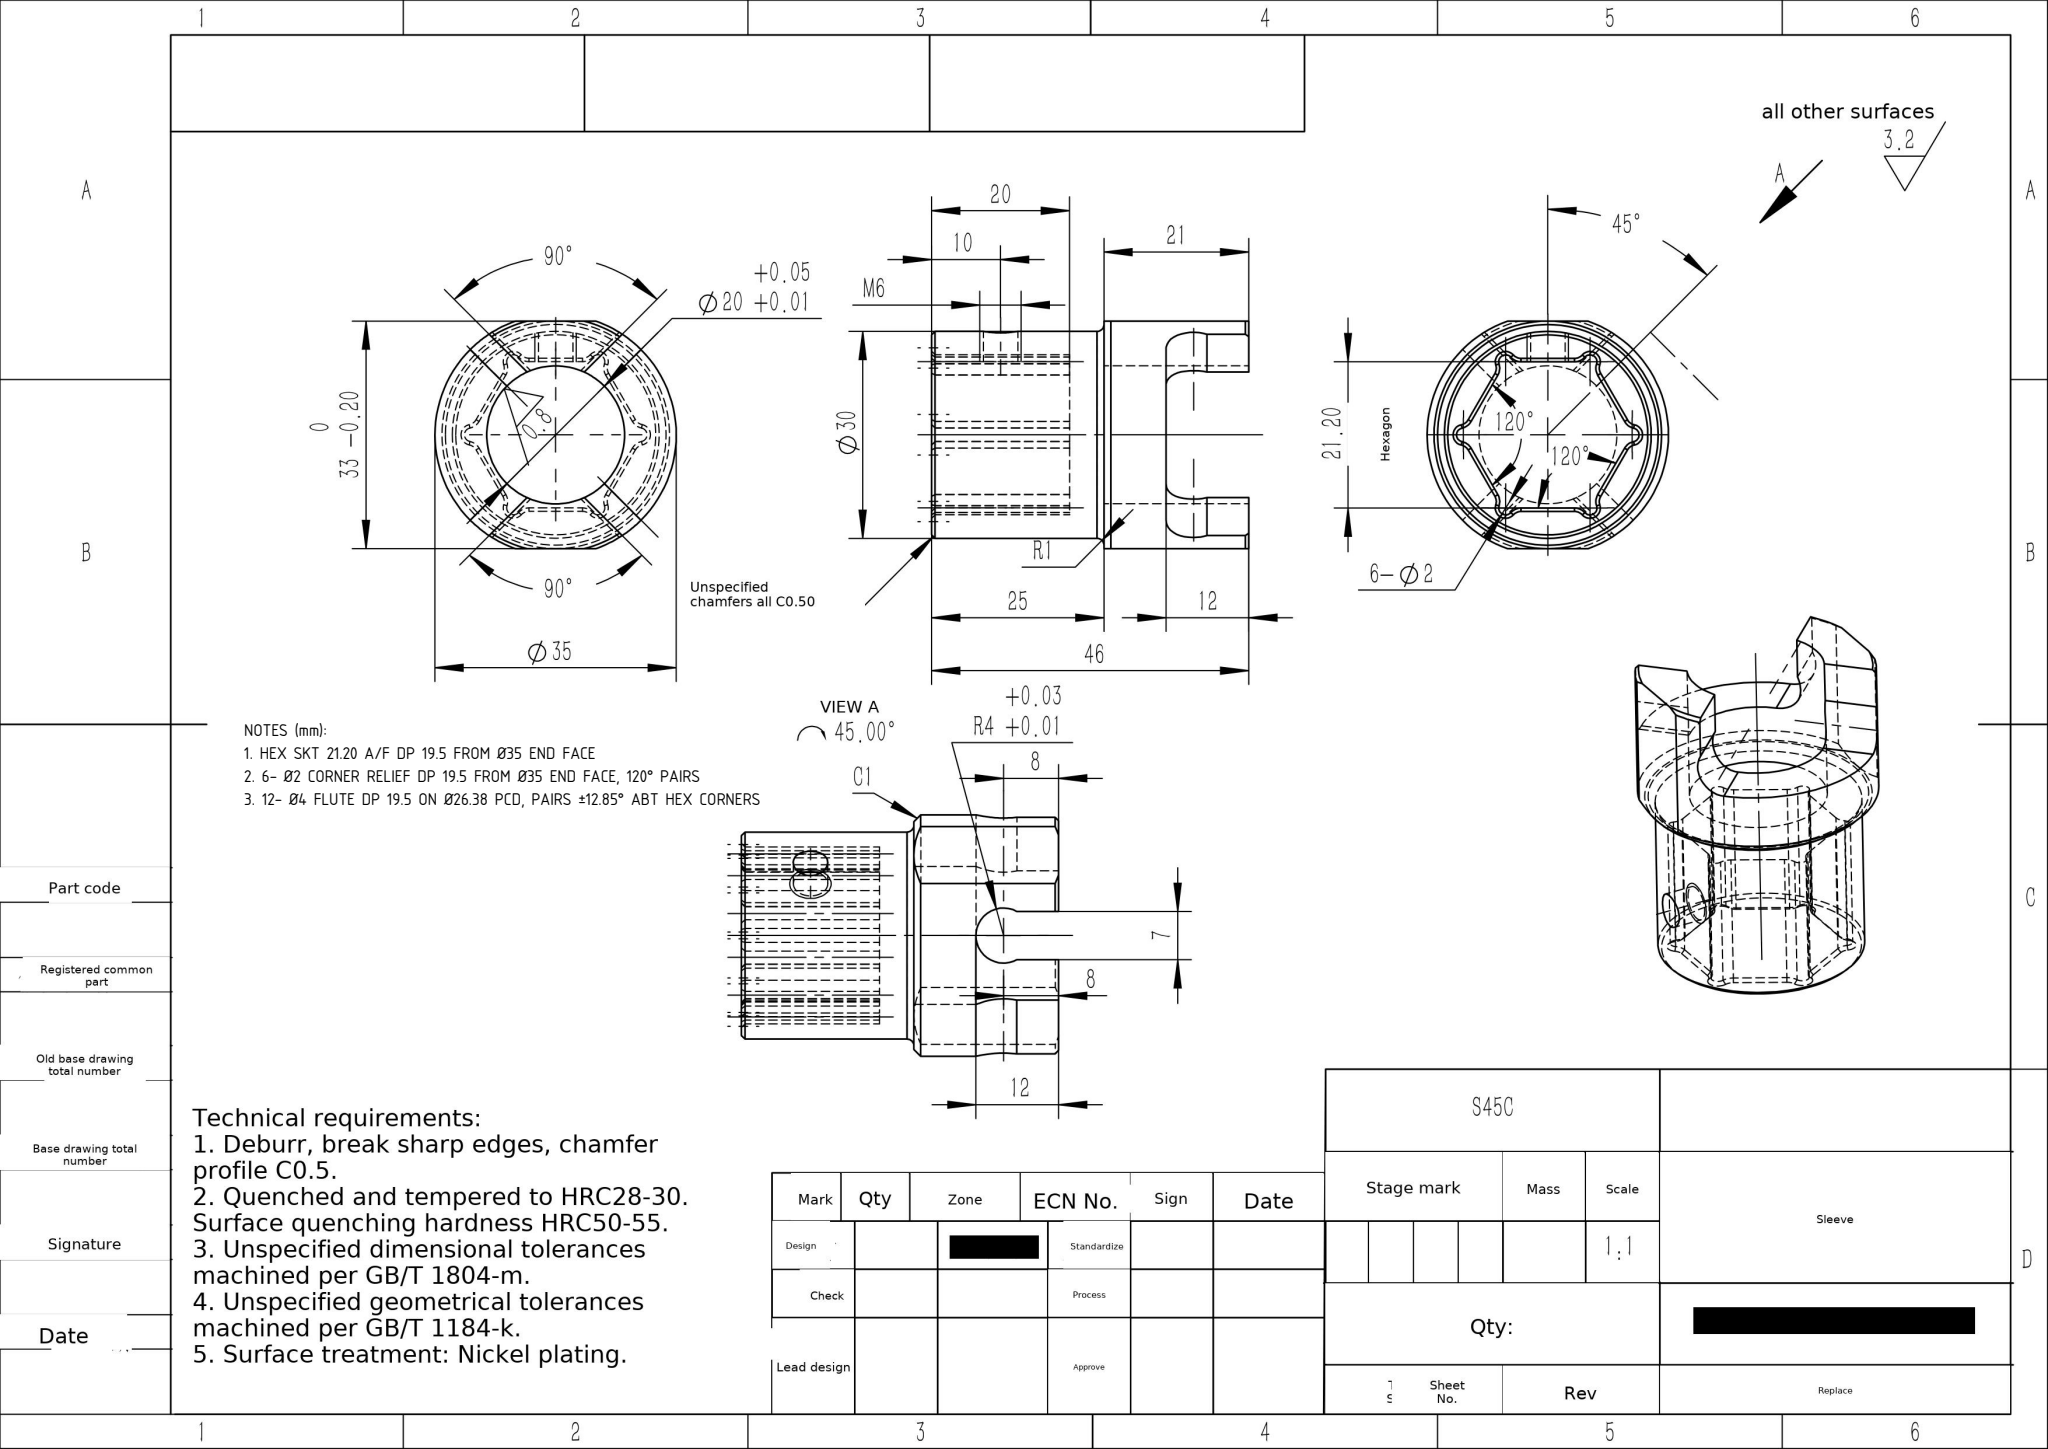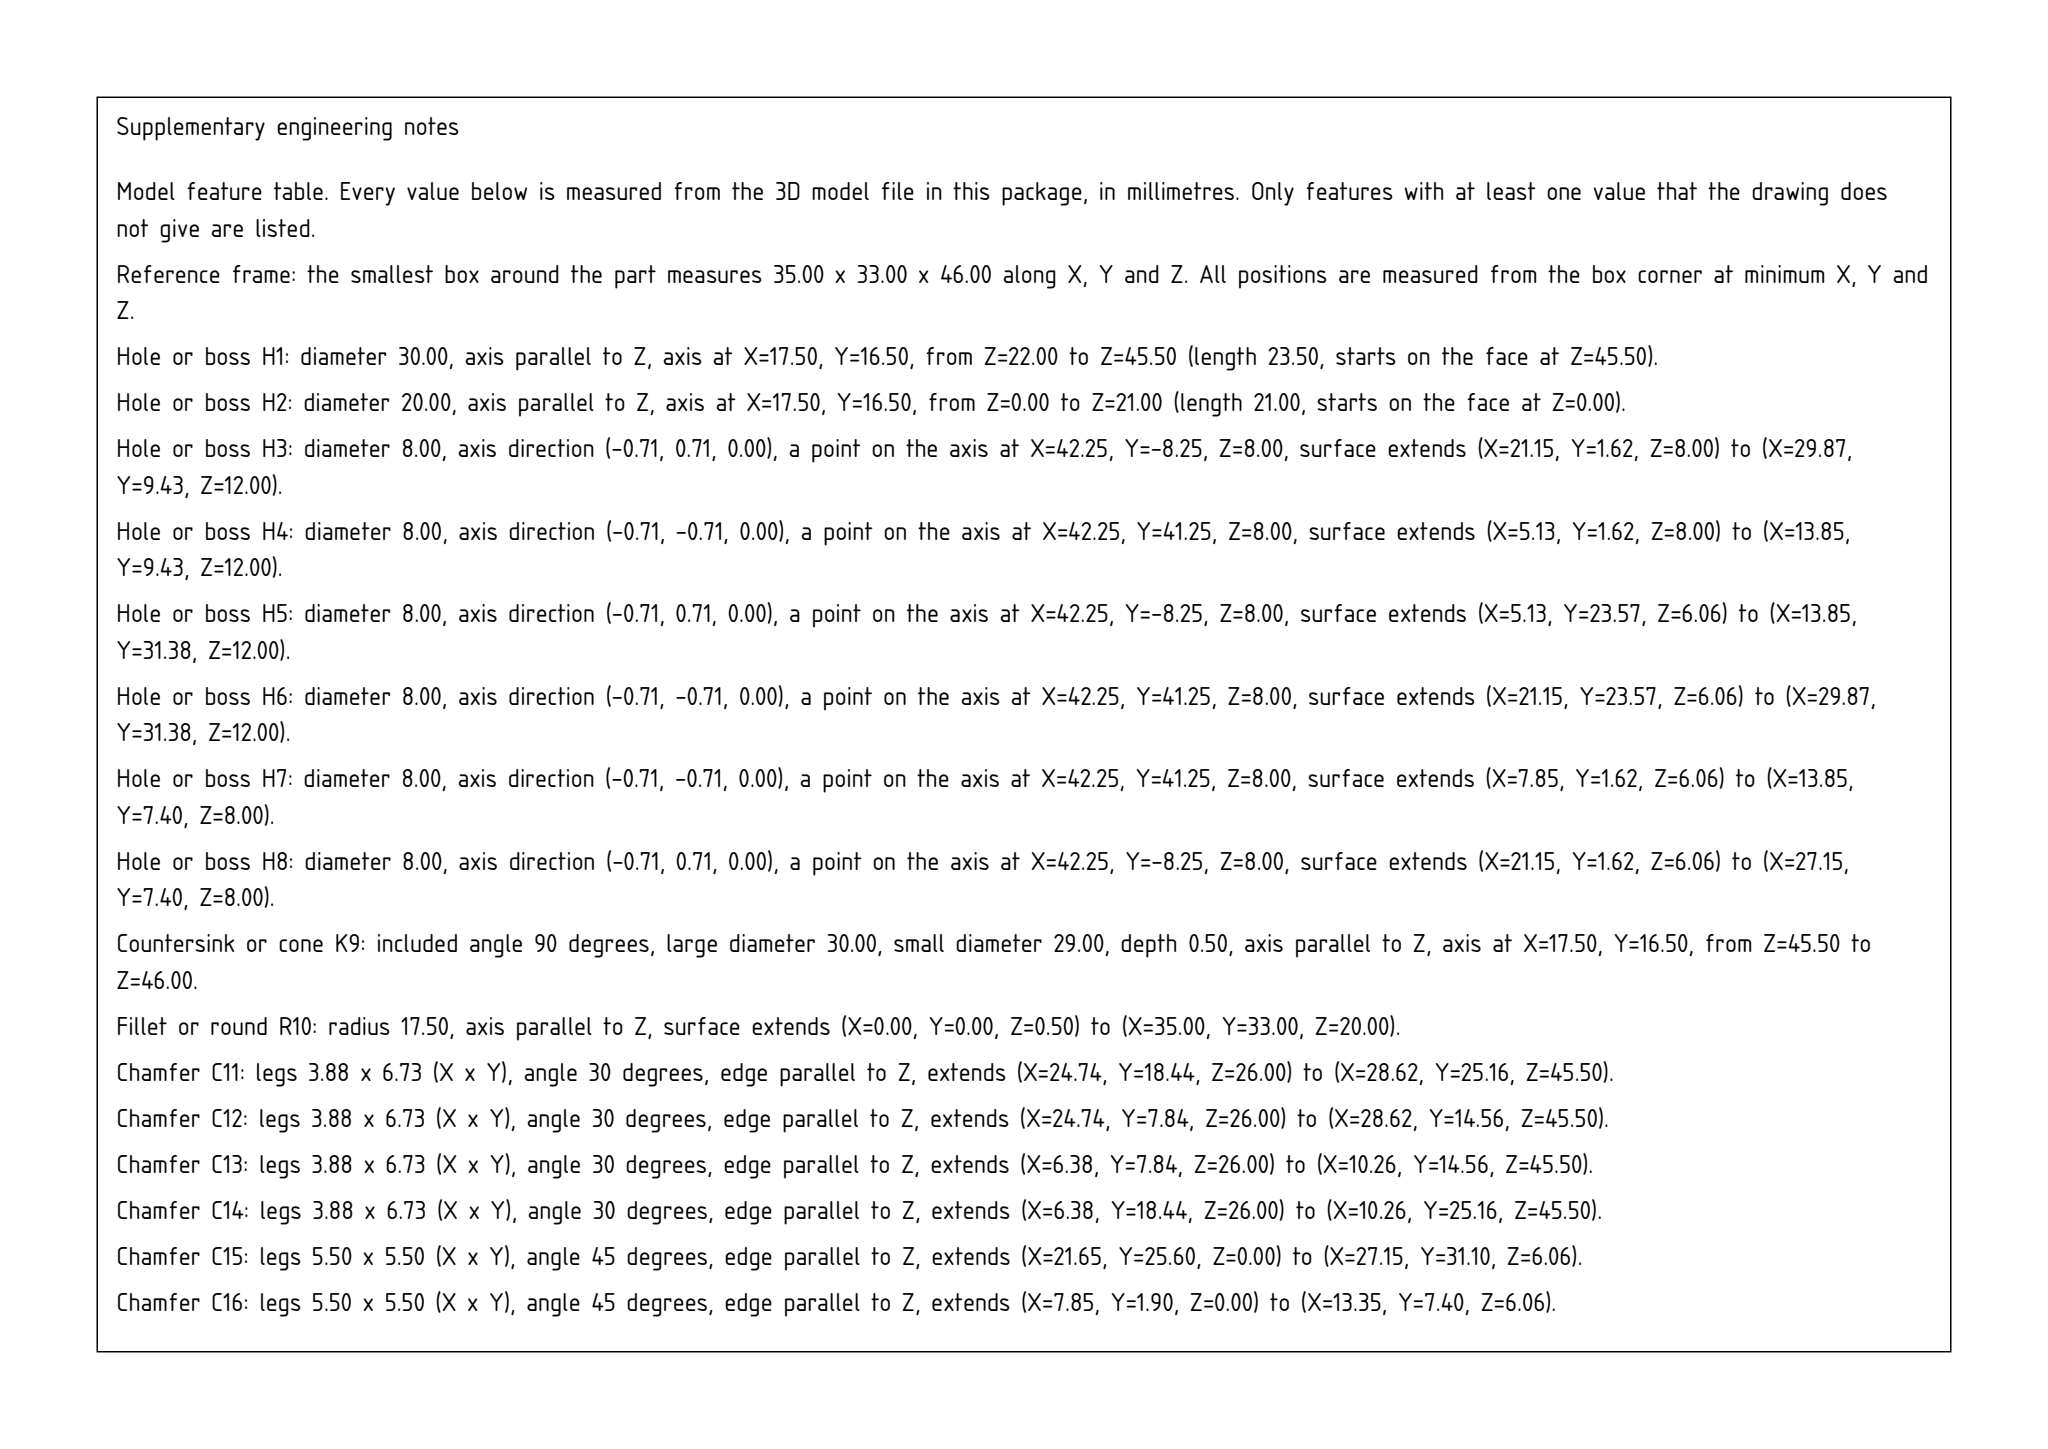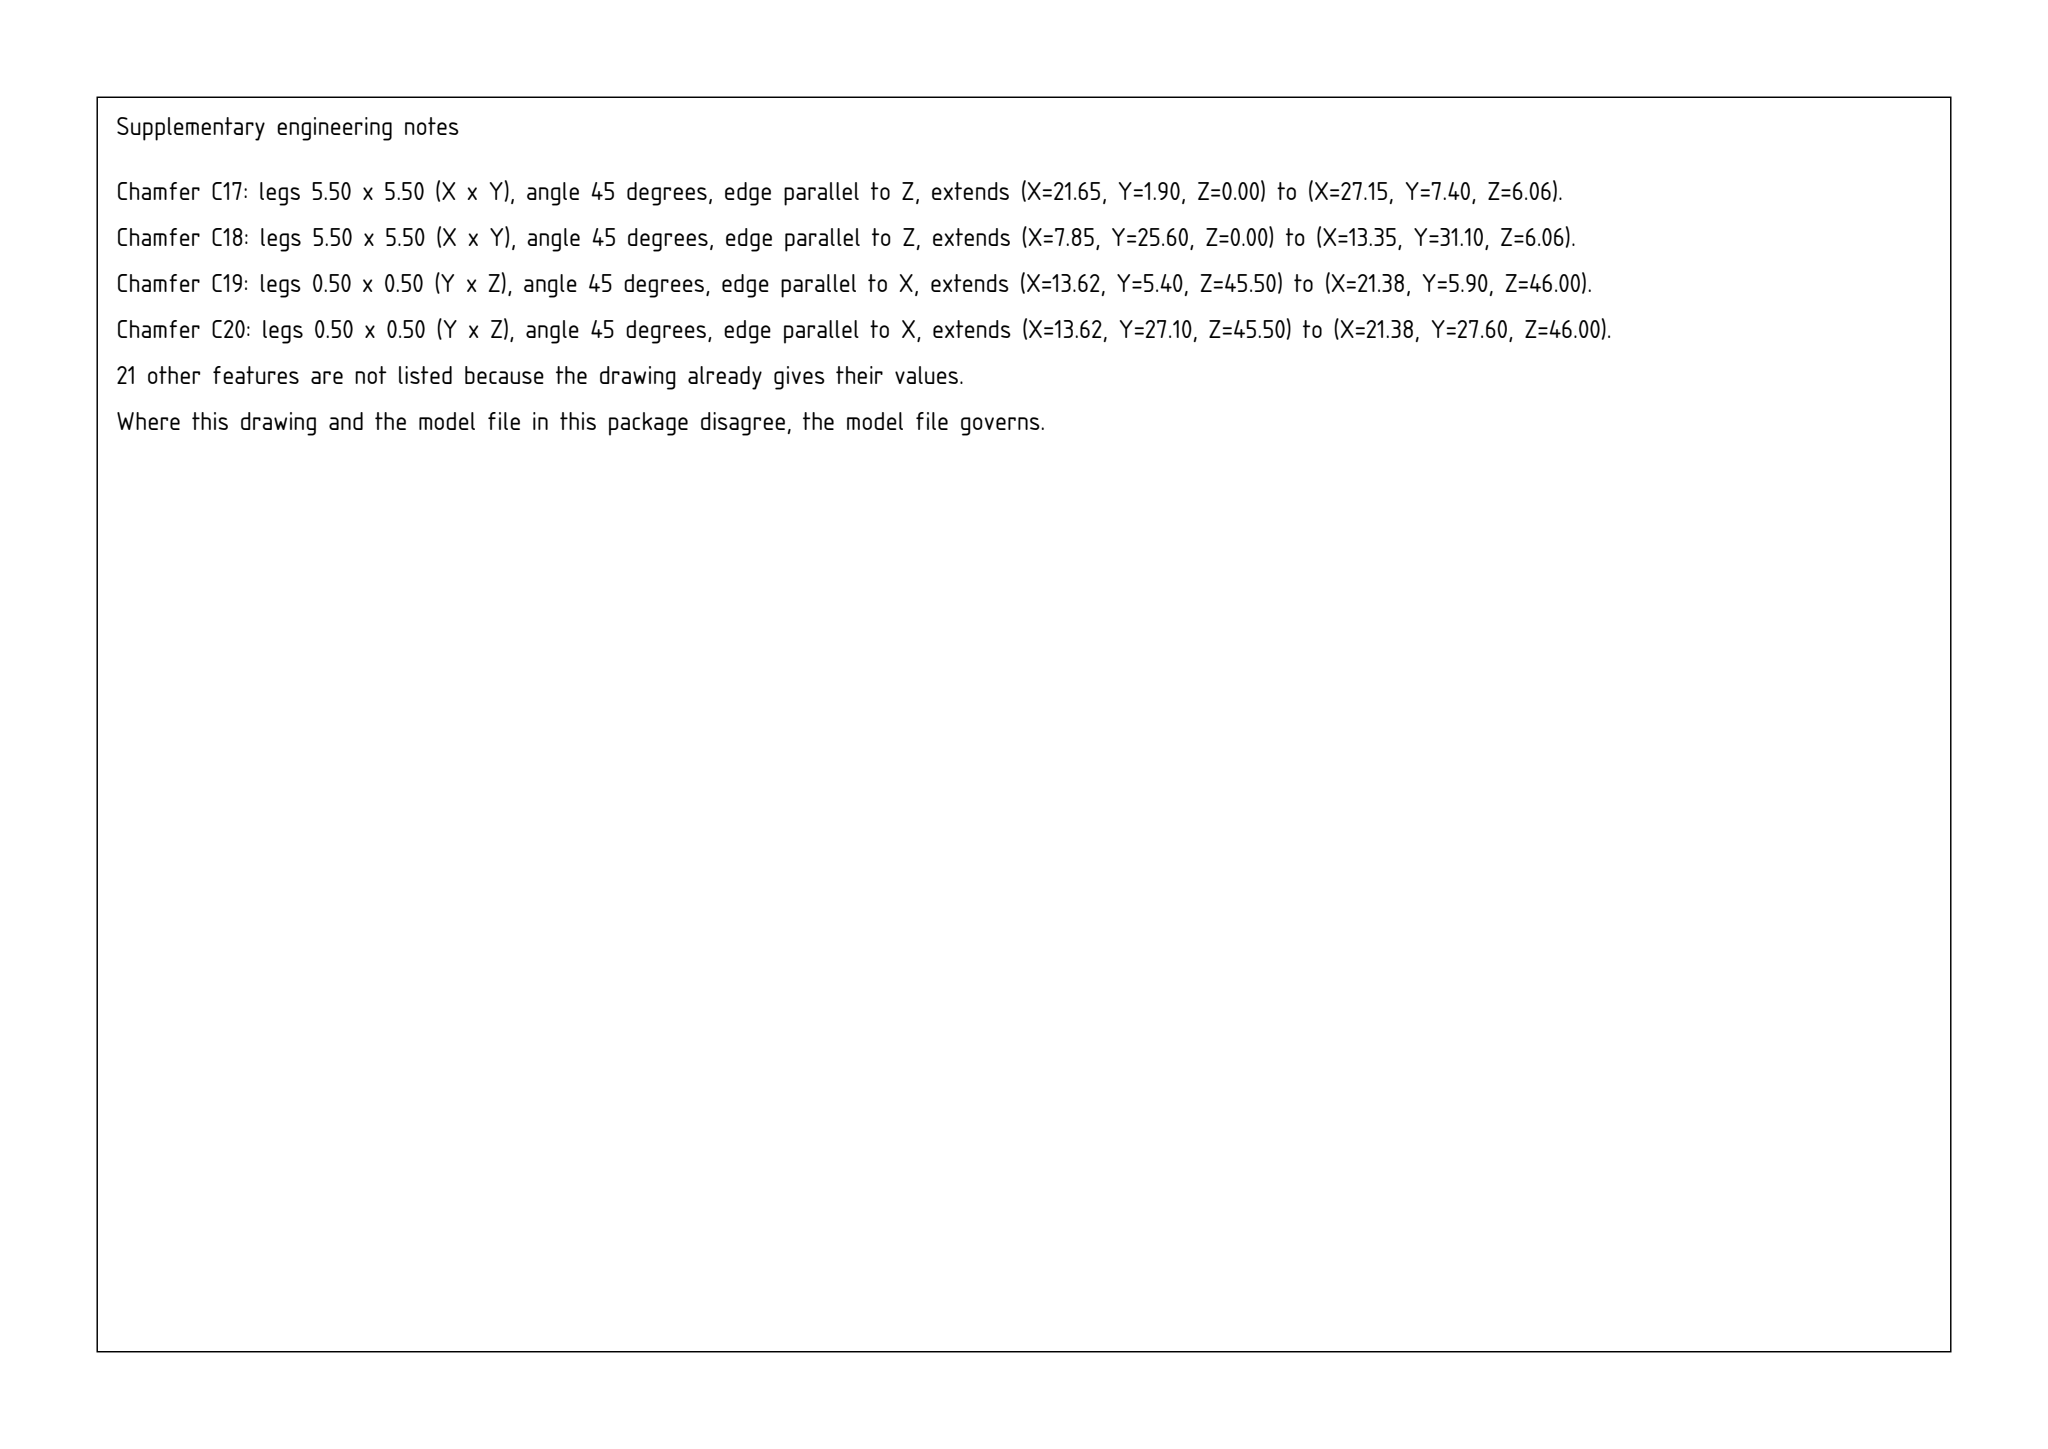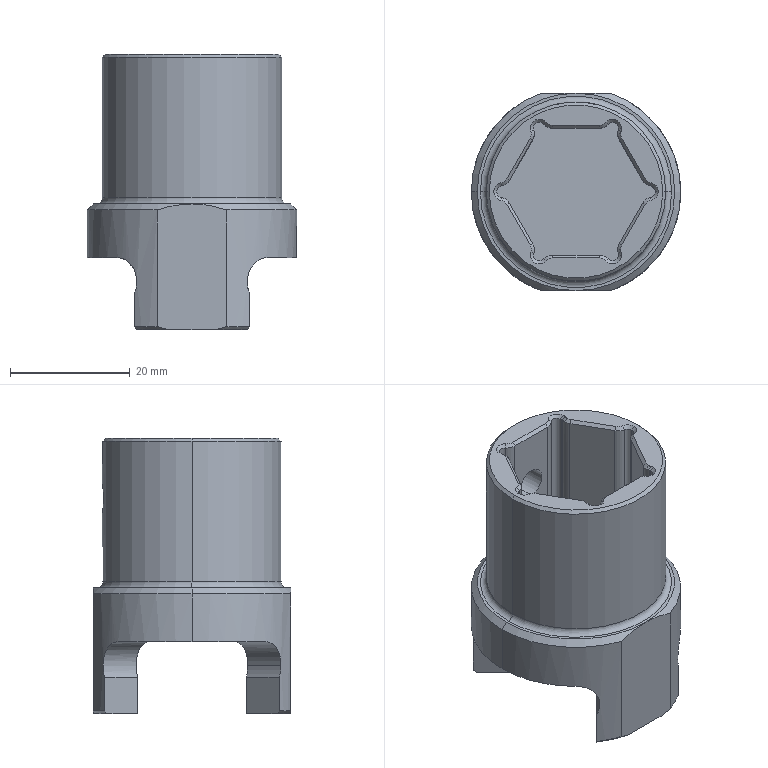Part | SolidWorks | mm | 1 solid | 98 faces | box 35 x 33 x 46 mm | volume 17595 mm3 | cylinder 38 | cone 32 | plane 26 | torus 2 | commonest cylinder face diameters 4 x14 2 x9 8 x6 35 x3 5 x2 30 x2 20 x2
Drawing notes:
HEX SKT 21.20 A/F DP 19.5 FROM Ø35 END FACE | from the solid: Hex corner holes/flutes all 19.5 long on z; Ø35 end face is hex-end datum; A/F from Ø2 corner holes at r12.24 (24.48 across corners x cos30 = 21.20)
6- Ø2 CORNER RELIEF DP 19.5 FROM Ø35 END FACE, 120° PAIRS | from the solid: 6x [2.0,'z',...,19.5] at (5.85,18.09),(11.97,7.49),(11.97,28.69),(24.21,7.49),(24.21,28.69),(30.33,18.09) about center (18.09,18.09), r=12.24
12- Ø4 FLUTE DP 19.5 ON Ø26.38 PCD, PAIRS ±12.85° ABT HEX CORNERS | from the solid: 12x [4.0,'z',...,19.5]; all at r=13.19 (PCD 26.38); angles 180±12.88, 240±12.88, 300±12.88, 0±12.88, 60±12.88, 120±12.88 = hex corner directions
build123d program:
from build123d import *

# Parameters (mm, degrees)
SKETCH1_R                     = 17.5
BOSS_EXTRUDE1_DEPTH           = 21
SKETCH2_R                     = 15
BOSS_EXTRUDE2_DEPTH           = 25
CHAMFER1_SIZE                 = 0.5
CHAMFER2_SIZE                 = 1
FILLET1_R                     = 1
CUT_EXTRUDE1_DEPTH            = 20
SKETCH4_R                     = 10
CUT_EXTRUDE2_DEPTH            = 21
SKETCH5_W                     = 25.734
SKETCH5_H                     = 2
SKETCH5_W_2                   = 26.658
CUT_EXTRUDE3_DEPTH            = 53.235
SKETCH6_R                     = 4
CUT_EXTRUDE4_DEPTH            = 50
CIRPATTERN1_COUNT             = 2
CIRPATTERN1_ANGLE             = 90
SKETCH7_W                     = 12.127
SKETCH7_H                     = 7
CUT_EXTRUDE5_DEPTH            = 50
CIRPATTERN2_COUNT             = 2
CIRPATTERN2_ANGLE             = 90
CUT_EXTRUDE6_DEPTH            = 12
SKETCH10_W                    = 2.5
SKETCH10_H                    = 15
SIZE_MM_DOWEL_PIN_HOLE1_D     = 2
SIZE_MM_DOWEL_PIN_HOLE1_DEPTH = 20
CIRPATTERN3_COUNT             = 6
FILLET2_R                     = 2
CHAMFER3_SIZE                 = 0.5


with BuildPart() as part:
    # Sketch1 → Boss-Extrude1 (new body)
    with BuildSketch(Plane.XY):
        with Locations(Location((0, 0, 0), (0, 0, 180))):
            Circle(SKETCH1_R)
    extrude(amount=BOSS_EXTRUDE1_DEPTH)

    # Sketch2 → Boss-Extrude2 (add)
    with BuildSketch(Plane.XY.offset(21)):
        Circle(SKETCH2_R)
    extrude(amount=BOSS_EXTRUDE2_DEPTH)

    # Chamfer1
    chamfer1_edges = [part.edges().sort_by_distance(p)[0] for p in [
        (17.5, 0, 0),
        (-15, 0, 46),
    ]]
    chamfer(chamfer1_edges, length=CHAMFER1_SIZE)

    # Chamfer2
    chamfer2_edges = [part.edges().sort_by_distance(p)[0] for p in [
        (17.5, 0, 21),
    ]]
    chamfer(chamfer2_edges, length=CHAMFER2_SIZE)

    # Fillet1
    fillet1_edges = [part.edges().sort_by_distance(p)[0] for p in [
        (-15, 0, 21),
    ]]
    fillet(fillet1_edges, radius=FILLET1_R)

    # Sketch3 → Cut-Extrude1 (cut)
    with BuildSketch(Plane.XY.offset(46)):
        Polygon((-6.12, 10.6), (-12.24, 0), (-6.12, -10.6), (6.12, -10.6), (12.24, 0), (6.12, 10.6), align=None)
    extrude(amount=-CUT_EXTRUDE1_DEPTH, mode=Mode.SUBTRACT)

    # Sketch4 → Cut-Extrude2 (cut)
    with BuildSketch(Plane(origin=(0, 0, 0), x_dir=(-1, 0, 0), z_dir=(0, 0, -1))):
        Circle(SKETCH4_R)
    extrude(amount=-CUT_EXTRUDE2_DEPTH, mode=Mode.SUBTRACT)

    # Sketch5 → Cut-Extrude3 (cut, through all)
    with BuildSketch(Plane(origin=(0, 0, 0), x_dir=(-1, 0, 0), z_dir=(0, 0, -1))):
        with Locations((0, -17.5)):
            Rectangle(SKETCH5_W, SKETCH5_H)
        with Locations((0, 17.5)):
            Rectangle(SKETCH5_W_2, SKETCH5_H)
    extrude(amount=-CUT_EXTRUDE3_DEPTH, mode=Mode.SUBTRACT)

    # Sketch6 → Cut-Extrude4 (cut, symmetric)
    with BuildSketch(Plane(origin=(-10.607, -10.607, 0), x_dir=(0, 0, -1), z_dir=(-0.7071, -0.7071, 0))):
        with Locations(Location((-8, 0, 0), (0, 0, 90))):
            Circle(SKETCH6_R)
    cut_extrude4 = extrude(amount=CUT_EXTRUDE4_DEPTH, both=True, mode=Mode.SUBTRACT)

    # CirPattern1: Cut-Extrude4 ×2 about axis
    cirpattern1_axis = Axis((0, 0, 0), (0, 0, 1))
    for i in range(1, CIRPATTERN1_COUNT):
        add(cut_extrude4.rotate(cirpattern1_axis, i * CIRPATTERN1_ANGLE / (CIRPATTERN1_COUNT - 1)), mode=Mode.SUBTRACT)

    # Sketch7 → Cut-Extrude5 (cut, symmetric)
    with BuildSketch(Plane(origin=(-10.607, -10.607, 0), x_dir=(0, 0, -1), z_dir=(-0.7071, -0.7071, 0))):
        Rectangle(SKETCH7_W, SKETCH7_H)
    cut_extrude5 = extrude(amount=CUT_EXTRUDE5_DEPTH, both=True, mode=Mode.SUBTRACT)

    # CirPattern2: Cut-Extrude5 ×2 about axis
    cirpattern2_axis = Axis((0, 0, 0.5), (0, 0, 1))
    for i in range(1, CIRPATTERN2_COUNT):
        add(cut_extrude5.rotate(cirpattern2_axis, i * CIRPATTERN2_ANGLE / (CIRPATTERN2_COUNT - 1)), mode=Mode.SUBTRACT)

    # Sketch8 → Cut-Extrude6 (cut)
    # profile 1 of 3: a face of its own
    with BuildSketch(Plane(origin=(0, 0, 0), x_dir=(-1, 0, 0), z_dir=(0, 0, -1))):
        Polygon((19.783, -19.783), (23.736, 23.736), (0, 0), align=None)
        with BuildLine():
            ThreePointArc((14.238, -9.288), (17, 0), (14.238, 9.288))
            Line((14.238, 9.288), (9.099, 4.149))
            ThreePointArc((9.099, 4.149), (10, 0), (9.099, -4.149))
            Line((9.099, -4.149), (14.238, -9.288))
        make_face(mode=Mode.SUBTRACT)
    # profile 2 of 3: a face of its own
    with BuildSketch(Plane(origin=(0, 0, 0), x_dir=(-1, 0, 0), z_dir=(0, 0, -1))):
        Polygon((-18.116, 18.116), (0, 0), (-18.116, -18.116), align=None)
    # profile 3 of 3: a face of its own
    with BuildSketch(Plane(origin=(0, 0, 0), x_dir=(-1, 0, 0), z_dir=(0, 0, -1))):
        with BuildLine():
            Line((9.099, -4.149), (14.238, -9.288))
            ThreePointArc((14.238, -9.288), (17, 0), (14.238, 9.288))
            Line((14.238, 9.288), (9.099, 4.149))
            ThreePointArc((9.099, 4.149), (10, 0), (9.099, -4.149))
        make_face()
    extrude(amount=-CUT_EXTRUDE6_DEPTH, mode=Mode.SUBTRACT)

    # Sketch10 → M6 Tapped Hole1 (revolve, cut)
    with BuildSketch(Plane(origin=(0, 0, 36), x_dir=(0, 0, -1), z_dir=(1, 0, 0))):
        with Locations((1.25, 7.5)):
            Rectangle(SKETCH10_W, SKETCH10_H)
    revolve(axis=Axis((0, -6.35, 36), (0, 1, 0)), mode=Mode.SUBTRACT)

    # Size mm Dowel Pin Hole1
    with Locations(Plane.XY.offset(46)):
        with Locations((12.24, 0)):
            size_mm_dowel_pin_hole1 = Hole(SIZE_MM_DOWEL_PIN_HOLE1_D / 2, depth=SIZE_MM_DOWEL_PIN_HOLE1_DEPTH)

    # CirPattern3: Size mm Dowel Pin Hole1 ×6 about axis
    cirpattern3_axis = Axis((0, 0, 0), (0, 0, 1))
    for i in range(1, CIRPATTERN3_COUNT):
        add(size_mm_dowel_pin_hole1.rotate(cirpattern3_axis, i * 360 / CIRPATTERN3_COUNT), mode=Mode.SUBTRACT)

    # Fillet2
    fillet2_edges = [part.edges().sort_by_distance(p)[0] for p in [
        (11.74, 0.866, 36),
        (11.74, -0.866, 36),
        (6.62, -9.734, 36),
        (5.12, -10.6, 36),
        (-5.12, -10.6, 36),
        (-6.62, -9.734, 36),
        (-11.74, -0.866, 36),
        (-11.74, 0.866, 36),
        (-5.12, 10.6, 36),
        (-6.62, 9.734, 36),
        (5.12, 10.6, 36),
        (6.62, 9.734, 36),
    ]]
    fillet(fillet2_edges, radius=FILLET2_R)

    # Chamfer3
    chamfer3_edges = [part.edges().sort_by_distance(p)[0] for p in [
        (0, 10.6, 46),
        (6.62, 11.466, 46),
        (9.18, 5.3, 46),
        (13.24, 0, 46),
        (9.18, -5.3, 46),
        (6.62, -11.466, 46),
        (0, -10.6, 46),
        (-6.62, -11.466, 46),
        (-9.18, -5.3, 46),
        (-13.24, 0, 46),
        (-9.18, 5.3, 46),
        (-6.62, 11.466, 46),
        (11.681, -1.317, 46),
        (6.981, 9.458, 46),
        (11.681, 1.317, 46),
        (6.981, -9.458, 46),
        (4.7, -10.774, 46),
        (-4.7, -10.774, 46),
        (-6.981, -9.458, 46),
        (-11.681, -1.317, 46),
        (-11.681, 1.317, 46),
        (-6.981, 9.458, 46),
        (-4.7, 10.774, 46),
        (4.7, 10.774, 46),
    ]]
    chamfer(chamfer3_edges, length=CHAMFER3_SIZE)


solid = part.part